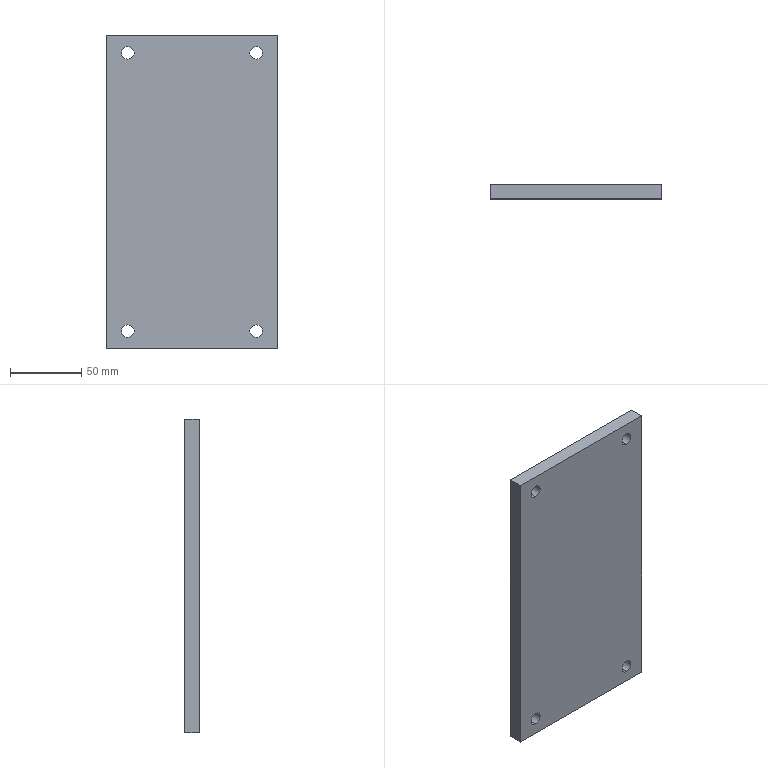Component | SolidWorks | MotorMount2-1 | 1 solid | 14 faces | box 120 x 10 x 220 mm | volume 261567 mm3 | cylinder 8 | plane 6 | commonest cylinder face diameters 8.8 x8
build123d program:
from build123d import *

# Parameters (mm, degrees)
SKETCH1_W                   = 220
SKETCH1_H                   = 120
EXTRUDE1_DEPTH              = 10
M10X1_25_TAPPED_HOLE1_D     = 8.8
M10X1_25_TAPPED_HOLE1_DEPTH = 26.25
M10X1_25_TAPPED_HOLE1_TIP   = 2.644


with BuildPart() as part:
    # Sketch1 → Extrude1 (new body)
    with BuildSketch(Plane.XY):
        with Locations((83.393, -39.305)):
            Rectangle(SKETCH1_W, SKETCH1_H)
    extrude(amount=EXTRUDE1_DEPTH)

    # M10x1.25 Tapped Hole1
    with Locations(Plane(origin=(-14.107, -84.305, 10), x_dir=(1, 0, 0), z_dir=(0, 0, 1))):
        with Locations((0, 0), (0, 90), (195, 90), (195, 0)):
            Hole(M10X1_25_TAPPED_HOLE1_D / 2, depth=M10X1_25_TAPPED_HOLE1_DEPTH)
            with Locations((0, 0, -(M10X1_25_TAPPED_HOLE1_DEPTH + M10X1_25_TAPPED_HOLE1_TIP / 2))):  # 118° drill point
                Cone(0, M10X1_25_TAPPED_HOLE1_D / 2, M10X1_25_TAPPED_HOLE1_TIP, mode=Mode.SUBTRACT)


solid = part.part

# Placed as in the assembly
solid = solid.moved(Location((-204.089, 106.983, -79.788), (90, 0, 90)))
STEP:
#1=COLOUR_RGB('',0.7922,0.8196,0.9333);
#2=FILL_AREA_STYLE_COLOUR('',#1);
#3=FILL_AREA_STYLE('',(#2));
#4=SURFACE_STYLE_FILL_AREA(#3);
#5=SURFACE_SIDE_STYLE('',(#4));
#6=SURFACE_STYLE_USAGE(.BOTH.,#5);
#7=PRESENTATION_STYLE_ASSIGNMENT((#6));
#8=CARTESIAN_POINT('',(-8.259,3.818,4.154));
#9=VERTEX_POINT('',#8);
#10=CARTESIAN_POINT('',(-8.259,3.818,3.807));
#11=VERTEX_POINT('',#10);
#12=CARTESIAN_POINT('',(-8.259,3.818,3.98));
#13=DIRECTION('',(0.,1.,-0.));
#14=DIRECTION('',(0.,0.,-1.));
#15=AXIS2_PLACEMENT_3D('',#12,#13,#14);
#16=CIRCLE('',#15,0.1732);
#17=EDGE_CURVE('',#9,#11,#16,.T.);
#18=ORIENTED_EDGE('',*,*,#17,.F.);
#19=CARTESIAN_POINT('',(-8.259,4.212,4.154));
#20=VERTEX_POINT('',#19);
#21=CARTESIAN_POINT('',(-8.259,4.212,4.154));
#22=DIRECTION('',(0.,1.,-0.));
#23=VECTOR('',#22,39.37);
#24=LINE('',#21,#23);
#25=EDGE_CURVE('',#9,#20,#24,.T.);
#26=ORIENTED_EDGE('',*,*,#25,.T.);
#27=CARTESIAN_POINT('',(-8.259,4.212,3.807));
#28=VERTEX_POINT('',#27);
#29=CARTESIAN_POINT('',(-8.259,4.212,3.98));
#30=DIRECTION('',(0.,1.,-0.));
#31=DIRECTION('',(0.,0.,-1.));
#32=AXIS2_PLACEMENT_3D('',#29,#30,#31);
#33=CIRCLE('',#32,0.1732);
#34=EDGE_CURVE('',#20,#28,#33,.T.);
#35=ORIENTED_EDGE('',*,*,#34,.T.);
#36=CARTESIAN_POINT('',(-8.259,4.212,3.807));
#37=DIRECTION('',(0.,1.,-0.));
#38=VECTOR('',#37,39.37);
#39=LINE('',#36,#38);
#40=EDGE_CURVE('',#11,#28,#39,.T.);
#41=ORIENTED_EDGE('',*,*,#40,.F.);
#42=EDGE_LOOP('',(#18,#26,#35,#41));
#43=FACE_OUTER_BOUND('',#42,.T.);
#44=CARTESIAN_POINT('',(-8.259,4.212,3.98));
#45=DIRECTION('',(0.,1.,-0.));
#46=DIRECTION('',(0.,0.,-1.));
#47=AXIS2_PLACEMENT_3D('',#44,#45,#46);
#48=CYLINDRICAL_SURFACE('',#47,0.1732);
#49=ADVANCED_FACE('',(#43),#48,.F.);
#50=CARTESIAN_POINT('',(-8.259,3.818,-3.523));
#51=VERTEX_POINT('',#50);
#52=CARTESIAN_POINT('',(-8.259,3.818,-3.87));
#53=VERTEX_POINT('',#52);
#54=CARTESIAN_POINT('',(-8.259,3.818,-3.697));
#55=DIRECTION('',(0.,1.,-0.));
#56=DIRECTION('',(0.,0.,-1.));
#57=AXIS2_PLACEMENT_3D('',#54,#55,#56);
#58=CIRCLE('',#57,0.1732);
#59=EDGE_CURVE('',#51,#53,#58,.T.);
#60=ORIENTED_EDGE('',*,*,#59,.F.);
#61=CARTESIAN_POINT('',(-8.259,4.212,-3.523));
#62=VERTEX_POINT('',#61);
#63=CARTESIAN_POINT('',(-8.259,4.212,-3.523));
#64=DIRECTION('',(0.,1.,-0.));
#65=VECTOR('',#64,39.37);
#66=LINE('',#63,#65);
#67=EDGE_CURVE('',#51,#62,#66,.T.);
#68=ORIENTED_EDGE('',*,*,#67,.T.);
#69=CARTESIAN_POINT('',(-8.259,4.212,-3.87));
#70=VERTEX_POINT('',#69);
#71=CARTESIAN_POINT('',(-8.259,4.212,-3.697));
#72=DIRECTION('',(0.,1.,-0.));
#73=DIRECTION('',(0.,0.,-1.));
#74=AXIS2_PLACEMENT_3D('',#71,#72,#73);
#75=CIRCLE('',#74,0.1732);
#76=EDGE_CURVE('',#62,#70,#75,.T.);
#77=ORIENTED_EDGE('',*,*,#76,.T.);
#78=CARTESIAN_POINT('',(-8.259,4.212,-3.87));
#79=DIRECTION('',(0.,1.,-0.));
#80=VECTOR('',#79,39.37);
#81=LINE('',#78,#80);
#82=EDGE_CURVE('',#53,#70,#81,.T.);
#83=ORIENTED_EDGE('',*,*,#82,.F.);
#84=EDGE_LOOP('',(#60,#68,#77,#83));
#85=FACE_OUTER_BOUND('',#84,.T.);
#86=CARTESIAN_POINT('',(-8.259,4.212,-3.697));
#87=DIRECTION('',(0.,1.,-0.));
#88=DIRECTION('',(0.,0.,-1.));
#89=AXIS2_PLACEMENT_3D('',#86,#87,#88);
#90=CYLINDRICAL_SURFACE('',#89,0.1732);
#91=ADVANCED_FACE('',(#85),#90,.F.);
#92=CARTESIAN_POINT('',(-4.716,3.818,-3.523));
#93=VERTEX_POINT('',#92);
#94=CARTESIAN_POINT('',(-4.716,3.818,-3.87));
#95=VERTEX_POINT('',#94);
#96=CARTESIAN_POINT('',(-4.716,3.818,-3.697));
#97=DIRECTION('',(0.,1.,-0.));
#98=DIRECTION('',(0.,0.,-1.));
#99=AXIS2_PLACEMENT_3D('',#96,#97,#98);
#100=CIRCLE('',#99,0.1732);
#101=EDGE_CURVE('',#93,#95,#100,.T.);
#102=ORIENTED_EDGE('',*,*,#101,.F.);
#103=CARTESIAN_POINT('',(-4.716,4.212,-3.523));
#104=VERTEX_POINT('',#103);
#105=CARTESIAN_POINT('',(-4.716,4.212,-3.523));
#106=DIRECTION('',(0.,1.,-0.));
#107=VECTOR('',#106,39.37);
#108=LINE('',#105,#107);
#109=EDGE_CURVE('',#93,#104,#108,.T.);
#110=ORIENTED_EDGE('',*,*,#109,.T.);
#111=CARTESIAN_POINT('',(-4.716,4.212,-3.87));
#112=VERTEX_POINT('',#111);
#113=CARTESIAN_POINT('',(-4.716,4.212,-3.697));
#114=DIRECTION('',(0.,1.,-0.));
#115=DIRECTION('',(0.,0.,-1.));
#116=AXIS2_PLACEMENT_3D('',#113,#114,#115);
#117=CIRCLE('',#116,0.1732);
#118=EDGE_CURVE('',#104,#112,#117,.T.);
#119=ORIENTED_EDGE('',*,*,#118,.T.);
#120=CARTESIAN_POINT('',(-4.716,4.212,-3.87));
#121=DIRECTION('',(0.,1.,-0.));
#122=VECTOR('',#121,39.37);
#123=LINE('',#120,#122);
#124=EDGE_CURVE('',#95,#112,#123,.T.);
#125=ORIENTED_EDGE('',*,*,#124,.F.);
#126=EDGE_LOOP('',(#102,#110,#119,#125));
#127=FACE_OUTER_BOUND('',#126,.T.);
#128=CARTESIAN_POINT('',(-4.716,4.212,-3.697));
#129=DIRECTION('',(0.,1.,-0.));
#130=DIRECTION('',(0.,0.,-1.));
#131=AXIS2_PLACEMENT_3D('',#128,#129,#130);
#132=CYLINDRICAL_SURFACE('',#131,0.1732);
#133=ADVANCED_FACE('',(#127),#132,.F.);
#134=CARTESIAN_POINT('',(-4.716,3.818,4.154));
#135=VERTEX_POINT('',#134);
#136=CARTESIAN_POINT('',(-4.716,3.818,3.807));
#137=VERTEX_POINT('',#136);
#138=CARTESIAN_POINT('',(-4.716,3.818,3.98));
#139=DIRECTION('',(0.,1.,-0.));
#140=DIRECTION('',(0.,0.,-1.));
#141=AXIS2_PLACEMENT_3D('',#138,#139,#140);
#142=CIRCLE('',#141,0.1732);
#143=EDGE_CURVE('',#135,#137,#142,.T.);
#144=ORIENTED_EDGE('',*,*,#143,.F.);
#145=CARTESIAN_POINT('',(-4.716,4.212,4.154));
#146=VERTEX_POINT('',#145);
#147=CARTESIAN_POINT('',(-4.716,4.212,4.154));
#148=DIRECTION('',(0.,1.,-0.));
#149=VECTOR('',#148,39.37);
#150=LINE('',#147,#149);
#151=EDGE_CURVE('',#135,#146,#150,.T.);
#152=ORIENTED_EDGE('',*,*,#151,.T.);
#153=CARTESIAN_POINT('',(-4.716,4.212,3.807));
#154=VERTEX_POINT('',#153);
#155=CARTESIAN_POINT('',(-4.716,4.212,3.98));
#156=DIRECTION('',(0.,1.,-0.));
#157=DIRECTION('',(0.,0.,-1.));
#158=AXIS2_PLACEMENT_3D('',#155,#156,#157);
#159=CIRCLE('',#158,0.1732);
#160=EDGE_CURVE('',#146,#154,#159,.T.);
#161=ORIENTED_EDGE('',*,*,#160,.T.);
#162=CARTESIAN_POINT('',(-4.716,4.212,3.807));
#163=DIRECTION('',(0.,1.,-0.));
#164=VECTOR('',#163,39.37);
#165=LINE('',#162,#164);
#166=EDGE_CURVE('',#137,#154,#165,.T.);
#167=ORIENTED_EDGE('',*,*,#166,.F.);
#168=EDGE_LOOP('',(#144,#152,#161,#167));
#169=FACE_OUTER_BOUND('',#168,.T.);
#170=CARTESIAN_POINT('',(-4.716,4.212,3.98));
#171=DIRECTION('',(0.,1.,-0.));
#172=DIRECTION('',(0.,0.,-1.));
#173=AXIS2_PLACEMENT_3D('',#170,#171,#172);
#174=CYLINDRICAL_SURFACE('',#173,0.1732);
#175=ADVANCED_FACE('',(#169),#174,.F.);
#176=CARTESIAN_POINT('',(-8.85,3.818,4.473));
#177=VERTEX_POINT('',#176);
#178=CARTESIAN_POINT('',(-4.125,3.818,4.473));
#179=VERTEX_POINT('',#178);
#180=CARTESIAN_POINT('',(-8.85,3.818,4.473));
#181=DIRECTION('',(1.,-0.,0.));
#182=VECTOR('',#181,39.37);
#183=LINE('',#180,#182);
#184=EDGE_CURVE('',#177,#179,#183,.T.);
#185=ORIENTED_EDGE('',*,*,#184,.T.);
#186=CARTESIAN_POINT('',(-4.125,4.212,4.473));
#187=VERTEX_POINT('',#186);
#188=CARTESIAN_POINT('',(-4.125,4.212,4.473));
#189=DIRECTION('',(-0.,-1.,0.));
#190=VECTOR('',#189,39.37);
#191=LINE('',#188,#190);
#192=EDGE_CURVE('',#187,#179,#191,.T.);
#193=ORIENTED_EDGE('',*,*,#192,.F.);
#194=CARTESIAN_POINT('',(-8.85,4.212,4.473));
#195=VERTEX_POINT('',#194);
#196=CARTESIAN_POINT('',(-8.85,4.212,4.473));
#197=DIRECTION('',(1.,-0.,0.));
#198=VECTOR('',#197,39.37);
#199=LINE('',#196,#198);
#200=EDGE_CURVE('',#195,#187,#199,.T.);
#201=ORIENTED_EDGE('',*,*,#200,.F.);
#202=CARTESIAN_POINT('',(-8.85,4.212,4.473));
#203=DIRECTION('',(-0.,-1.,0.));
#204=VECTOR('',#203,39.37);
#205=LINE('',#202,#204);
#206=EDGE_CURVE('',#195,#177,#205,.T.);
#207=ORIENTED_EDGE('',*,*,#206,.T.);
#208=EDGE_LOOP('',(#185,#193,#201,#207));
#209=FACE_OUTER_BOUND('',#208,.T.);
#210=CARTESIAN_POINT('',(-8.85,4.212,4.473));
#211=DIRECTION('',(0.,-0.,-1.));
#212=DIRECTION('',(-1.,0.,-0.));
#213=AXIS2_PLACEMENT_3D('',#210,#211,#212);
#214=PLANE('',#213);
#215=ADVANCED_FACE('',(#209),#214,.F.);
#216=CARTESIAN_POINT('',(-4.125,3.818,-4.189));
#217=VERTEX_POINT('',#216);
#218=CARTESIAN_POINT('',(-4.125,3.818,4.473));
#219=DIRECTION('',(0.,-0.,-1.));
#220=VECTOR('',#219,39.37);
#221=LINE('',#218,#220);
#222=EDGE_CURVE('',#179,#217,#221,.T.);
#223=ORIENTED_EDGE('',*,*,#222,.T.);
#224=CARTESIAN_POINT('',(-4.125,4.212,-4.189));
#225=VERTEX_POINT('',#224);
#226=CARTESIAN_POINT('',(-4.125,4.212,-4.189));
#227=DIRECTION('',(-0.,-1.,0.));
#228=VECTOR('',#227,39.37);
#229=LINE('',#226,#228);
#230=EDGE_CURVE('',#225,#217,#229,.T.);
#231=ORIENTED_EDGE('',*,*,#230,.F.);
#232=CARTESIAN_POINT('',(-4.125,4.212,4.473));
#233=DIRECTION('',(0.,-0.,-1.));
#234=VECTOR('',#233,39.37);
#235=LINE('',#232,#234);
#236=EDGE_CURVE('',#187,#225,#235,.T.);
#237=ORIENTED_EDGE('',*,*,#236,.F.);
#238=ORIENTED_EDGE('',*,*,#192,.T.);
#239=EDGE_LOOP('',(#223,#231,#237,#238));
#240=FACE_OUTER_BOUND('',#239,.T.);
#241=CARTESIAN_POINT('',(-4.125,4.212,4.473));
#242=DIRECTION('',(-1.,0.,-0.));
#243=DIRECTION('',(0.,1.,-0.));
#244=AXIS2_PLACEMENT_3D('',#241,#242,#243);
#245=PLANE('',#244);
#246=ADVANCED_FACE('',(#240),#245,.F.);
#247=CARTESIAN_POINT('',(-8.85,3.818,-4.189));
#248=VERTEX_POINT('',#247);
#249=CARTESIAN_POINT('',(-8.85,3.818,-4.189));
#250=DIRECTION('',(-1.,0.,-0.));
#251=VECTOR('',#250,39.37);
#252=LINE('',#249,#251);
#253=EDGE_CURVE('',#217,#248,#252,.T.);
#254=ORIENTED_EDGE('',*,*,#253,.T.);
#255=CARTESIAN_POINT('',(-8.85,4.212,-4.189));
#256=VERTEX_POINT('',#255);
#257=CARTESIAN_POINT('',(-8.85,4.212,-4.189));
#258=DIRECTION('',(-0.,-1.,0.));
#259=VECTOR('',#258,39.37);
#260=LINE('',#257,#259);
#261=EDGE_CURVE('',#256,#248,#260,.T.);
#262=ORIENTED_EDGE('',*,*,#261,.F.);
#263=CARTESIAN_POINT('',(-8.85,4.212,-4.189));
#264=DIRECTION('',(-1.,0.,-0.));
#265=VECTOR('',#264,39.37);
#266=LINE('',#263,#265);
#267=EDGE_CURVE('',#225,#256,#266,.T.);
#268=ORIENTED_EDGE('',*,*,#267,.F.);
#269=ORIENTED_EDGE('',*,*,#230,.T.);
#270=EDGE_LOOP('',(#254,#262,#268,#269));
#271=FACE_OUTER_BOUND('',#270,.T.);
#272=CARTESIAN_POINT('',(-8.85,4.212,-4.189));
#273=DIRECTION('',(-0.,0.,1.));
#274=DIRECTION('',(1.,-0.,0.));
#275=AXIS2_PLACEMENT_3D('',#272,#273,#274);
#276=PLANE('',#275);
#277=ADVANCED_FACE('',(#271),#276,.F.);
#278=CARTESIAN_POINT('',(-8.85,3.818,4.473));
#279=DIRECTION('',(-0.,0.,1.));
#280=VECTOR('',#279,39.37);
#281=LINE('',#278,#280);
#282=EDGE_CURVE('',#248,#177,#281,.T.);
#283=ORIENTED_EDGE('',*,*,#282,.T.);
#284=ORIENTED_EDGE('',*,*,#206,.F.);
#285=CARTESIAN_POINT('',(-8.85,4.212,4.473));
#286=DIRECTION('',(-0.,0.,1.));
#287=VECTOR('',#286,39.37);
#288=LINE('',#285,#287);
#289=EDGE_CURVE('',#256,#195,#288,.T.);
#290=ORIENTED_EDGE('',*,*,#289,.F.);
#291=ORIENTED_EDGE('',*,*,#261,.T.);
#292=EDGE_LOOP('',(#283,#284,#290,#291));
#293=FACE_OUTER_BOUND('',#292,.T.);
#294=CARTESIAN_POINT('',(-8.85,4.212,4.473));
#295=DIRECTION('',(1.,-0.,0.));
#296=DIRECTION('',(-0.,-1.,0.));
#297=AXIS2_PLACEMENT_3D('',#294,#295,#296);
#298=PLANE('',#297);
#299=ADVANCED_FACE('',(#293),#298,.F.);
#300=CARTESIAN_POINT('',(-8.259,4.212,3.98));
#301=DIRECTION('',(0.,1.,-0.));
#302=DIRECTION('',(0.,0.,-1.));
#303=AXIS2_PLACEMENT_3D('',#300,#301,#302);
#304=CIRCLE('',#303,0.1732);
#305=EDGE_CURVE('',#28,#20,#304,.T.);
#306=ORIENTED_EDGE('',*,*,#305,.F.);
#307=ORIENTED_EDGE('',*,*,#34,.F.);
#308=EDGE_LOOP('',(#306,#307));
#309=FACE_BOUND('',#308,.T.);
#310=CARTESIAN_POINT('',(-8.259,4.212,-3.697));
#311=DIRECTION('',(0.,1.,-0.));
#312=DIRECTION('',(0.,0.,-1.));
#313=AXIS2_PLACEMENT_3D('',#310,#311,#312);
#314=CIRCLE('',#313,0.1732);
#315=EDGE_CURVE('',#70,#62,#314,.T.);
#316=ORIENTED_EDGE('',*,*,#315,.F.);
#317=ORIENTED_EDGE('',*,*,#76,.F.);
#318=EDGE_LOOP('',(#316,#317));
#319=FACE_BOUND('',#318,.T.);
#320=CARTESIAN_POINT('',(-4.716,4.212,-3.697));
#321=DIRECTION('',(0.,1.,-0.));
#322=DIRECTION('',(0.,0.,-1.));
#323=AXIS2_PLACEMENT_3D('',#320,#321,#322);
#324=CIRCLE('',#323,0.1732);
#325=EDGE_CURVE('',#112,#104,#324,.T.);
#326=ORIENTED_EDGE('',*,*,#325,.F.);
#327=ORIENTED_EDGE('',*,*,#118,.F.);
#328=EDGE_LOOP('',(#326,#327));
#329=FACE_BOUND('',#328,.T.);
#330=CARTESIAN_POINT('',(-4.716,4.212,3.98));
#331=DIRECTION('',(0.,1.,-0.));
#332=DIRECTION('',(0.,0.,-1.));
#333=AXIS2_PLACEMENT_3D('',#330,#331,#332);
#334=CIRCLE('',#333,0.1732);
#335=EDGE_CURVE('',#154,#146,#334,.T.);
#336=ORIENTED_EDGE('',*,*,#335,.F.);
#337=ORIENTED_EDGE('',*,*,#160,.F.);
#338=EDGE_LOOP('',(#336,#337));
#339=FACE_BOUND('',#338,.T.);
#340=ORIENTED_EDGE('',*,*,#200,.T.);
#341=ORIENTED_EDGE('',*,*,#236,.T.);
#342=ORIENTED_EDGE('',*,*,#267,.T.);
#343=ORIENTED_EDGE('',*,*,#289,.T.);
#344=EDGE_LOOP('',(#340,#341,#342,#343));
#345=FACE_OUTER_BOUND('',#344,.T.);
#346=CARTESIAN_POINT('',(-4.125,4.212,4.473));
#347=DIRECTION('',(0.,1.,-0.));
#348=DIRECTION('',(0.,-0.,-1.));
#349=AXIS2_PLACEMENT_3D('',#346,#347,#348);
#350=PLANE('',#349);
#351=ADVANCED_FACE('',(#309,#319,#329,#339,#345),#350,.T.);
#352=CARTESIAN_POINT('',(-8.259,3.818,3.98));
#353=DIRECTION('',(0.,1.,-0.));
#354=DIRECTION('',(0.,0.,-1.));
#355=AXIS2_PLACEMENT_3D('',#352,#353,#354);
#356=CIRCLE('',#355,0.1732);
#357=EDGE_CURVE('',#11,#9,#356,.T.);
#358=ORIENTED_EDGE('',*,*,#357,.T.);
#359=ORIENTED_EDGE('',*,*,#17,.T.);
#360=EDGE_LOOP('',(#358,#359));
#361=FACE_BOUND('',#360,.T.);
#362=CARTESIAN_POINT('',(-8.259,3.818,-3.697));
#363=DIRECTION('',(0.,1.,-0.));
#364=DIRECTION('',(0.,0.,-1.));
#365=AXIS2_PLACEMENT_3D('',#362,#363,#364);
#366=CIRCLE('',#365,0.1732);
#367=EDGE_CURVE('',#53,#51,#366,.T.);
#368=ORIENTED_EDGE('',*,*,#367,.T.);
#369=ORIENTED_EDGE('',*,*,#59,.T.);
#370=EDGE_LOOP('',(#368,#369));
#371=FACE_BOUND('',#370,.T.);
#372=CARTESIAN_POINT('',(-4.716,3.818,-3.697));
#373=DIRECTION('',(0.,1.,-0.));
#374=DIRECTION('',(0.,0.,-1.));
#375=AXIS2_PLACEMENT_3D('',#372,#373,#374);
#376=CIRCLE('',#375,0.1732);
#377=EDGE_CURVE('',#95,#93,#376,.T.);
#378=ORIENTED_EDGE('',*,*,#377,.T.);
#379=ORIENTED_EDGE('',*,*,#101,.T.);
#380=EDGE_LOOP('',(#378,#379));
#381=FACE_BOUND('',#380,.T.);
#382=CARTESIAN_POINT('',(-4.716,3.818,3.98));
#383=DIRECTION('',(0.,1.,-0.));
#384=DIRECTION('',(0.,0.,-1.));
#385=AXIS2_PLACEMENT_3D('',#382,#383,#384);
#386=CIRCLE('',#385,0.1732);
#387=EDGE_CURVE('',#137,#135,#386,.T.);
#388=ORIENTED_EDGE('',*,*,#387,.T.);
#389=ORIENTED_EDGE('',*,*,#143,.T.);
#390=EDGE_LOOP('',(#388,#389));
#391=FACE_BOUND('',#390,.T.);
#392=ORIENTED_EDGE('',*,*,#184,.F.);
#393=ORIENTED_EDGE('',*,*,#282,.F.);
#394=ORIENTED_EDGE('',*,*,#253,.F.);
#395=ORIENTED_EDGE('',*,*,#222,.F.);
#396=EDGE_LOOP('',(#392,#393,#394,#395));
#397=FACE_OUTER_BOUND('',#396,.T.);
#398=CARTESIAN_POINT('',(-4.125,3.818,4.473));
#399=DIRECTION('',(0.,1.,-0.));
#400=DIRECTION('',(0.,-0.,-1.));
#401=AXIS2_PLACEMENT_3D('',#398,#399,#400);
#402=PLANE('',#401);
#403=ADVANCED_FACE('',(#361,#371,#381,#391,#397),#402,.F.);
#404=ORIENTED_EDGE('',*,*,#151,.F.);
#405=ORIENTED_EDGE('',*,*,#387,.F.);
#406=ORIENTED_EDGE('',*,*,#166,.T.);
#407=ORIENTED_EDGE('',*,*,#335,.T.);
#408=EDGE_LOOP('',(#404,#405,#406,#407));
#409=FACE_OUTER_BOUND('',#408,.T.);
#410=CARTESIAN_POINT('',(-4.716,4.212,3.98));
#411=DIRECTION('',(0.,1.,-0.));
#412=DIRECTION('',(0.,0.,-1.));
#413=AXIS2_PLACEMENT_3D('',#410,#411,#412);
#414=CYLINDRICAL_SURFACE('',#413,0.1732);
#415=ADVANCED_FACE('',(#409),#414,.F.);
#416=ORIENTED_EDGE('',*,*,#109,.F.);
#417=ORIENTED_EDGE('',*,*,#377,.F.);
#418=ORIENTED_EDGE('',*,*,#124,.T.);
#419=ORIENTED_EDGE('',*,*,#325,.T.);
#420=EDGE_LOOP('',(#416,#417,#418,#419));
#421=FACE_OUTER_BOUND('',#420,.T.);
#422=CARTESIAN_POINT('',(-4.716,4.212,-3.697));
#423=DIRECTION('',(0.,1.,-0.));
#424=DIRECTION('',(0.,0.,-1.));
#425=AXIS2_PLACEMENT_3D('',#422,#423,#424);
#426=CYLINDRICAL_SURFACE('',#425,0.1732);
#427=ADVANCED_FACE('',(#421),#426,.F.);
#428=ORIENTED_EDGE('',*,*,#67,.F.);
#429=ORIENTED_EDGE('',*,*,#367,.F.);
#430=ORIENTED_EDGE('',*,*,#82,.T.);
#431=ORIENTED_EDGE('',*,*,#315,.T.);
#432=EDGE_LOOP('',(#428,#429,#430,#431));
#433=FACE_OUTER_BOUND('',#432,.T.);
#434=CARTESIAN_POINT('',(-8.259,4.212,-3.697));
#435=DIRECTION('',(0.,1.,-0.));
#436=DIRECTION('',(0.,0.,-1.));
#437=AXIS2_PLACEMENT_3D('',#434,#435,#436);
#438=CYLINDRICAL_SURFACE('',#437,0.1732);
#439=ADVANCED_FACE('',(#433),#438,.F.);
#440=ORIENTED_EDGE('',*,*,#25,.F.);
#441=ORIENTED_EDGE('',*,*,#357,.F.);
#442=ORIENTED_EDGE('',*,*,#40,.T.);
#443=ORIENTED_EDGE('',*,*,#305,.T.);
#444=EDGE_LOOP('',(#440,#441,#442,#443));
#445=FACE_OUTER_BOUND('',#444,.T.);
#446=CARTESIAN_POINT('',(-8.259,4.212,3.98));
#447=DIRECTION('',(0.,1.,-0.));
#448=DIRECTION('',(0.,0.,-1.));
#449=AXIS2_PLACEMENT_3D('',#446,#447,#448);
#450=CYLINDRICAL_SURFACE('',#449,0.1732);
#451=ADVANCED_FACE('',(#445),#450,.F.);
#452=CLOSED_SHELL('',(#49,#91,#133,#175,#215,#246,#277,#299,#351,#403,#415,#427,#439,#451));
#453=MANIFOLD_SOLID_BREP('',#452);
#454=STYLED_ITEM('',(#7),#453);
#455=PRESENTATION_LAYER_ASSIGNMENT('','',(#454));
#456=CARTESIAN_POINT('',(0.,0.,0.));
#457=DIRECTION('',(0.,0.,1.));
#458=DIRECTION('',(1.,0.,0.));
#459=AXIS2_PLACEMENT_3D('',#456,#457,#458);
#460=(LENGTH_UNIT()NAMED_UNIT(*)SI_UNIT($,.METRE.));
#461=LENGTH_MEASURE_WITH_UNIT(LENGTH_MEASURE(0.0254),#460);
#462=DIMENSIONAL_EXPONENTS(1.,0.,0.,0.,0.,0.,0.);
#463=(CONVERSION_BASED_UNIT('',#461)LENGTH_UNIT()NAMED_UNIT(#462));
#464=UNCERTAINTY_MEASURE_WITH_UNIT(LENGTH_MEASURE(0.00001),#463,'','');
#465=(NAMED_UNIT(*)PLANE_ANGLE_UNIT()SI_UNIT($,.RADIAN.));
#466=(NAMED_UNIT(*)SI_UNIT($,.STERADIAN.)SOLID_ANGLE_UNIT());
#467=(GEOMETRIC_REPRESENTATION_CONTEXT(3)GLOBAL_UNCERTAINTY_ASSIGNED_CONTEXT((#464))GLOBAL_UNIT_ASSIGNED_CONTEXT((#463,#465,#466))REPRESENTATION_CONTEXT('',''));
#468=ADVANCED_BREP_SHAPE_REPRESENTATION('',(#453,#459),#467);
#469=(LENGTH_UNIT()NAMED_UNIT(*)SI_UNIT($,.METRE.));
#470=LENGTH_MEASURE_WITH_UNIT(LENGTH_MEASURE(0.0254),#469);
#471=DIMENSIONAL_EXPONENTS(1.,0.,0.,0.,0.,0.,0.);
#472=(CONVERSION_BASED_UNIT('',#470)LENGTH_UNIT()NAMED_UNIT(#471));
#473=UNCERTAINTY_MEASURE_WITH_UNIT(LENGTH_MEASURE(0.00001),#472,'','');
#474=(NAMED_UNIT(*)PLANE_ANGLE_UNIT()SI_UNIT($,.RADIAN.));
#475=(NAMED_UNIT(*)SI_UNIT($,.STERADIAN.)SOLID_ANGLE_UNIT());
#476=(GEOMETRIC_REPRESENTATION_CONTEXT(3)GLOBAL_UNCERTAINTY_ASSIGNED_CONTEXT((#473))GLOBAL_UNIT_ASSIGNED_CONTEXT((#472,#474,#475))REPRESENTATION_CONTEXT('',''));
#477=MECHANICAL_DESIGN_GEOMETRIC_PRESENTATION_REPRESENTATION('',(#454),#476);